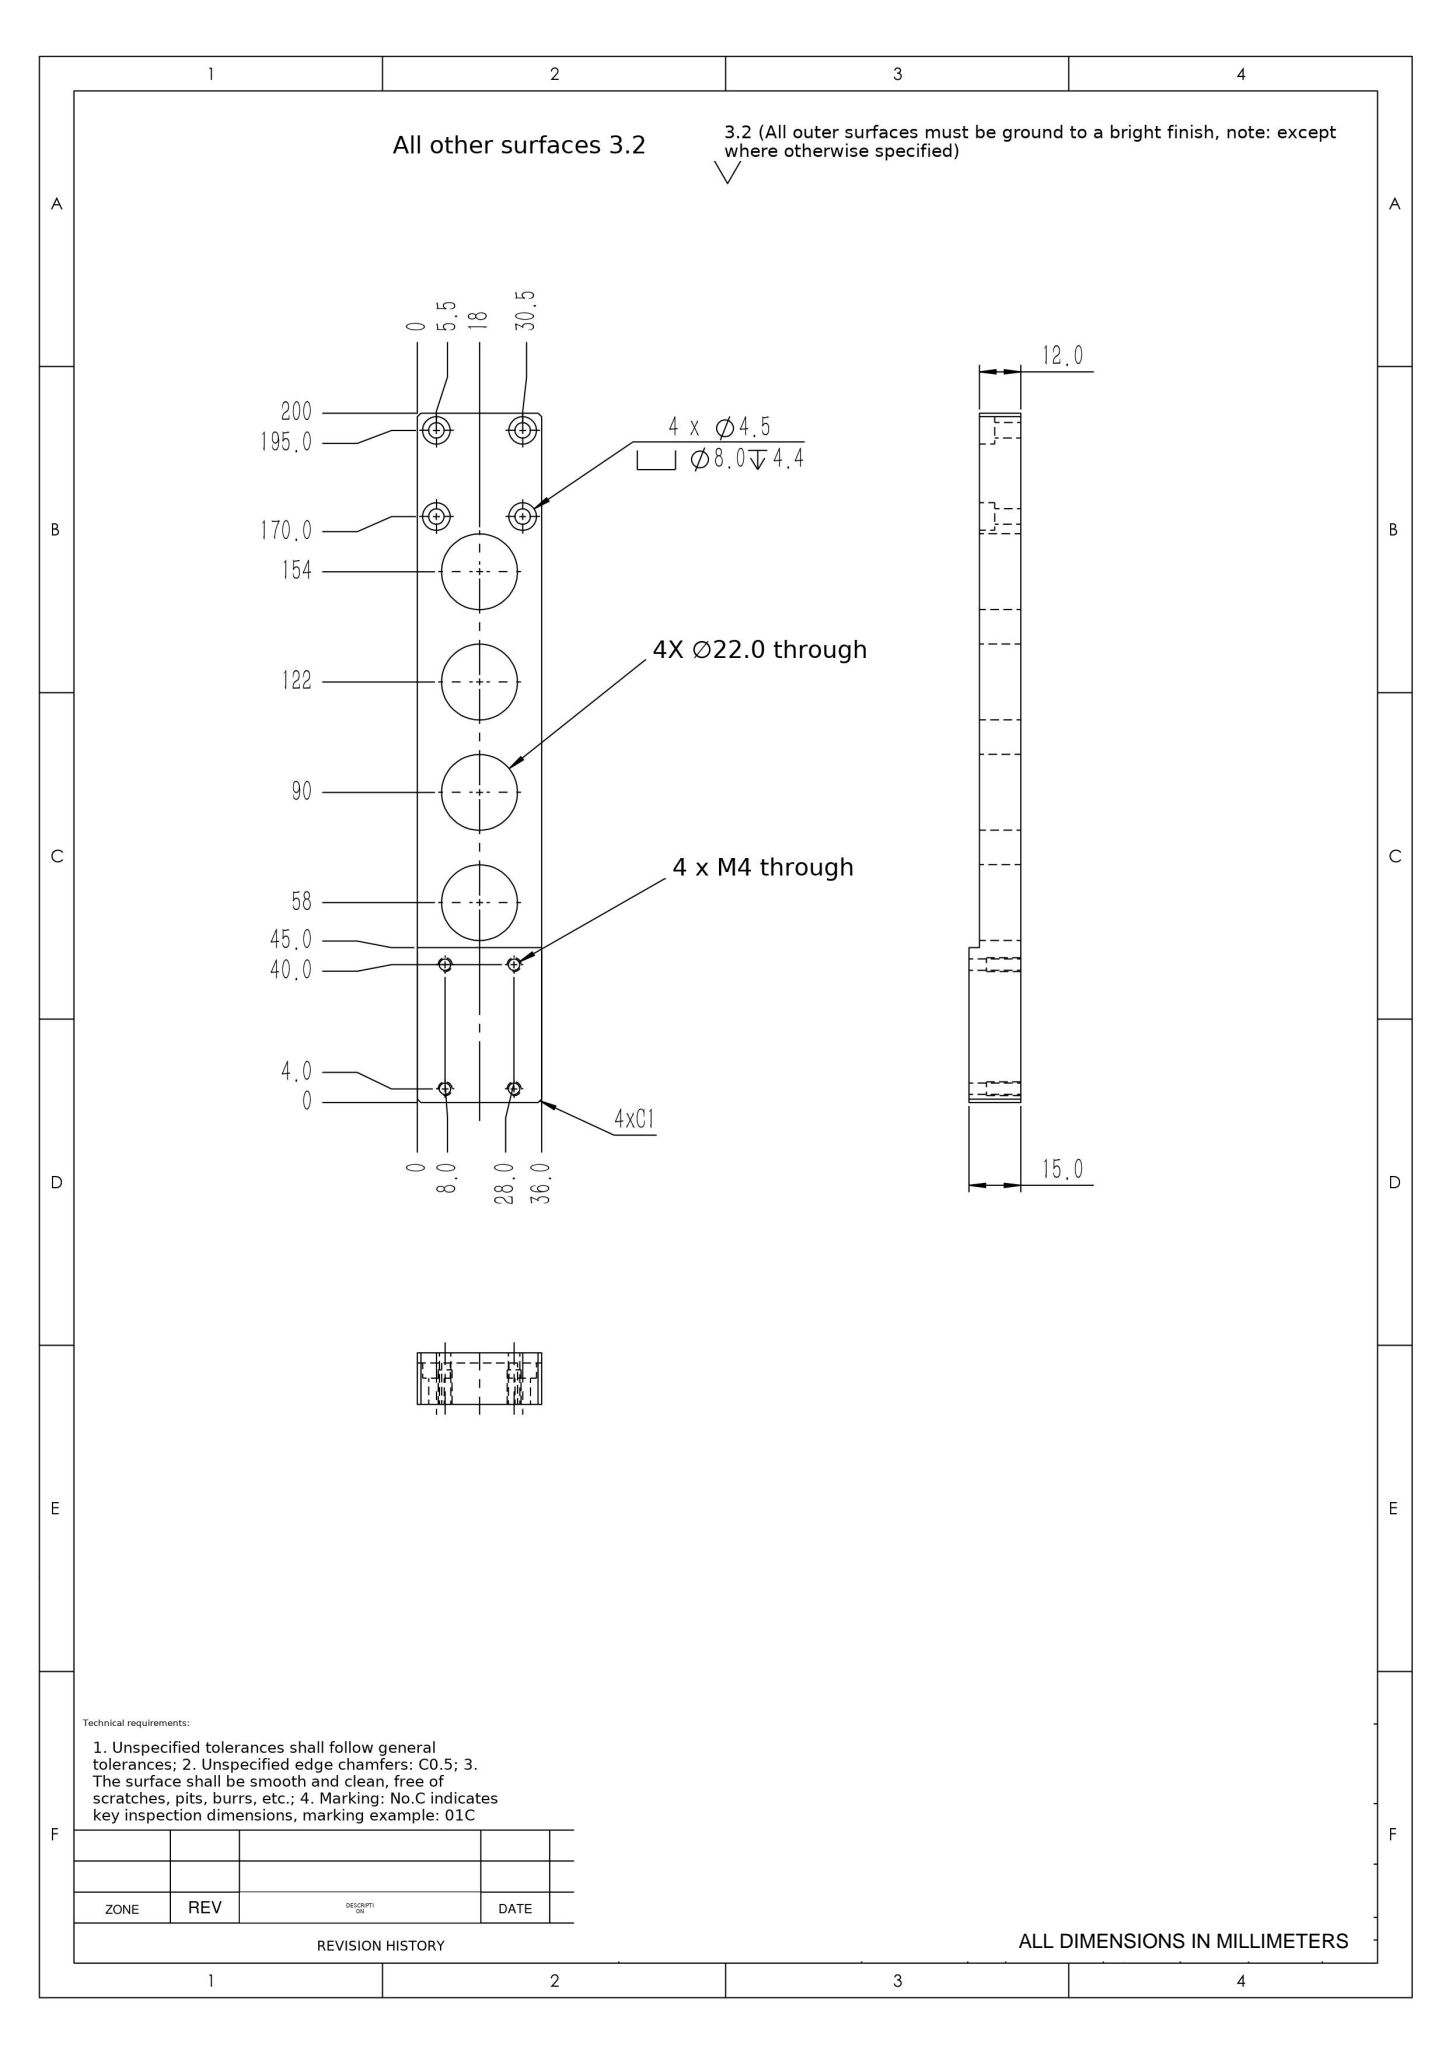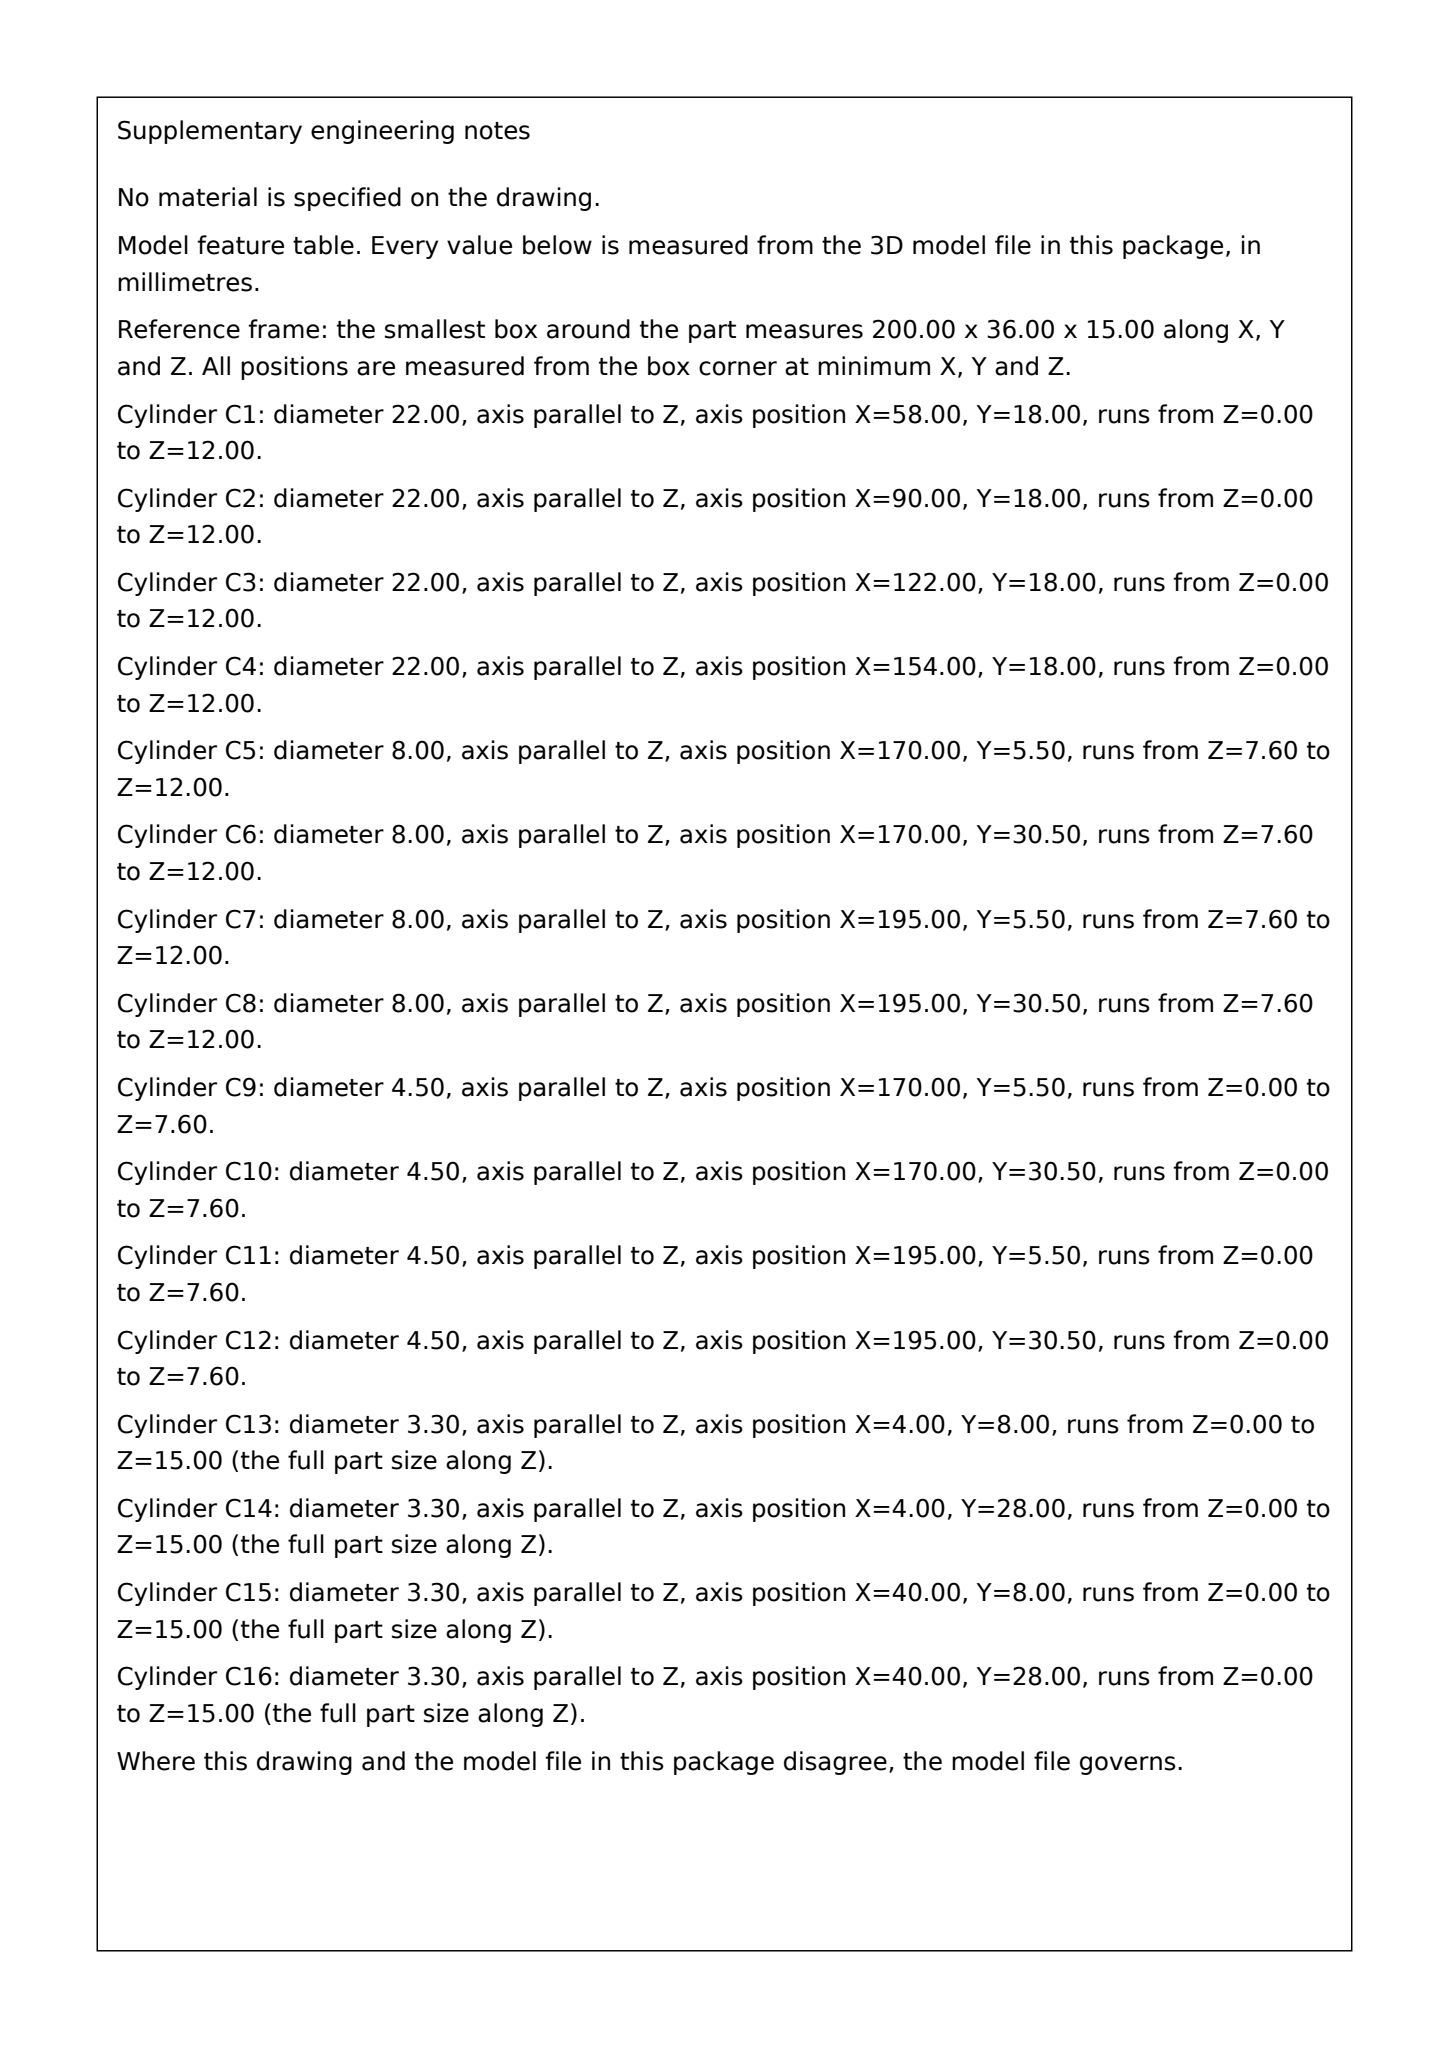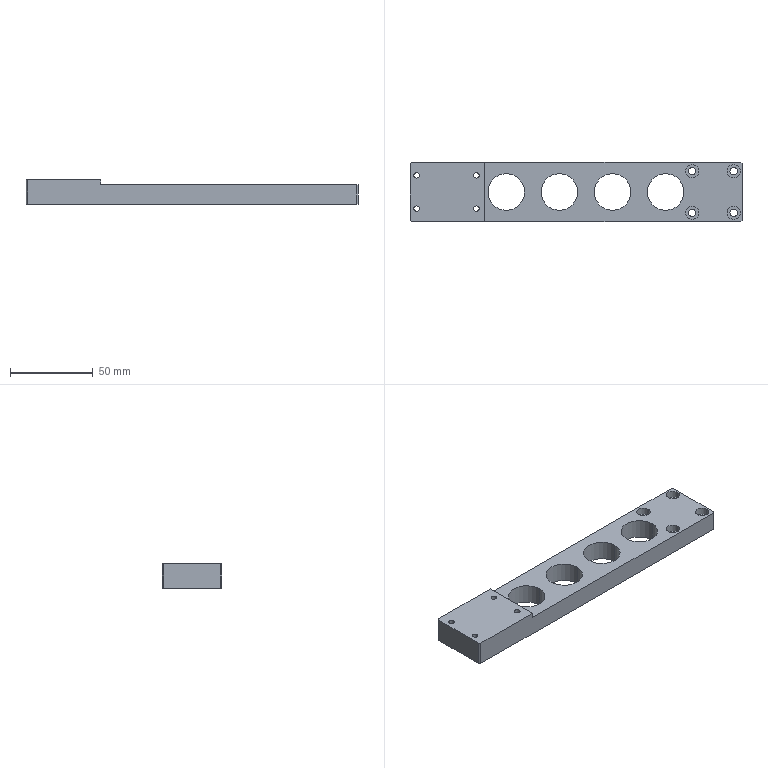Part | SolidWorks | mm | 1 solid | 48 faces | box 200 x 36 x 15 mm | volume 71105 mm3 | cylinder 32 | plane 16 | commonest cylinder face diameters 22 x8 3.3 x8 8 x8 4.5 x8
build123d program:
from build123d import *

# Parameters (mm, degrees)
SKETCH1_W                                       = 200
SKETCH1_H                                       = 36
BOSS_EXTRUDE1_DEPTH                             = 6
M4_HEX_SOCKET_HEAD_CAP_SCREW_CBORE1_D           = 4.5
M4_HEX_SOCKET_HEAD_CAP_SCREW_CBORE1_CBORE_D     = 8
M4_HEX_SOCKET_HEAD_CAP_SCREW_CBORE1_CBORE_DEPTH = 4.4
CHAMFER1_SIZE                                   = 1
SKETCH8_W                                       = 45
SKETCH8_H                                       = 36
BOSS_EXTRUDE2_DEPTH                             = 3
M4_TAPPED_HOLE1_D                               = 3.3
CHAMFER2_SIZE                                   = 1
SKETCH7_R                                       = 11
CUT_EXTRUDE2_DEPTH                              = 103.313
LPATTERN1_COUNT                                 = 4
LPATTERN1_PITCH                                 = 32


with BuildPart() as part:
    # Sketch1 → Boss-Extrude1 (new, symmetric)
    with BuildSketch(Plane.XY):
        Rectangle(SKETCH1_W, SKETCH1_H)
    extrude(amount=BOSS_EXTRUDE1_DEPTH, both=True)

    # M4 Hex Socket Head Cap Screw CBORE1 (through all)
    with Locations(Plane.XY.offset(6)):
        with Locations((95, 12.5), (95, -12.5), (70, -12.5), (70, 12.5)):
            CounterBoreHole(M4_HEX_SOCKET_HEAD_CAP_SCREW_CBORE1_D / 2, M4_HEX_SOCKET_HEAD_CAP_SCREW_CBORE1_CBORE_D / 2, M4_HEX_SOCKET_HEAD_CAP_SCREW_CBORE1_CBORE_DEPTH)

    # Chamfer1
    chamfer1_edges = [part.edges().sort_by_distance(p)[0] for p in [
        (100, -18, 0),
        (100, 18, 0),
    ]]
    chamfer(chamfer1_edges, length=CHAMFER1_SIZE)

    # Sketch8 → Boss-Extrude2 (add)
    with BuildSketch(Plane.XY.offset(6)):
        with Locations((-77.5, 0)):
            Rectangle(SKETCH8_W, SKETCH8_H)
    extrude(amount=BOSS_EXTRUDE2_DEPTH)

    # M4 Tapped Hole1 (through all)
    with Locations(Plane(origin=(0, 0, -6), x_dir=(-1, 0, 0), z_dir=(0, 0, -1))):
        with Locations((96, 10), (96, -10), (60, -10), (60, 10)):
            Hole(M4_TAPPED_HOLE1_D / 2)

    # Chamfer2
    chamfer2_edges = [part.edges().sort_by_distance(p)[0] for p in [
        (-100, -18, 1.5),
        (-100, 18, 1.5),
    ]]
    chamfer(chamfer2_edges, length=CHAMFER2_SIZE)

    # Sketch7 → Cut-Extrude2 (cut, through all)
    with BuildSketch(Plane.XY.offset(6)):
        with Locations((-42, 0)):
            Circle(SKETCH7_R)
    cut_extrude2 = extrude(amount=-CUT_EXTRUDE2_DEPTH, mode=Mode.SUBTRACT)

    # LPattern1: Cut-Extrude2 ×4
    with Locations(*[(i * LPATTERN1_PITCH, 0, 0) for i in range(1, LPATTERN1_COUNT)]):
        add(cut_extrude2, mode=Mode.SUBTRACT)


solid = part.part